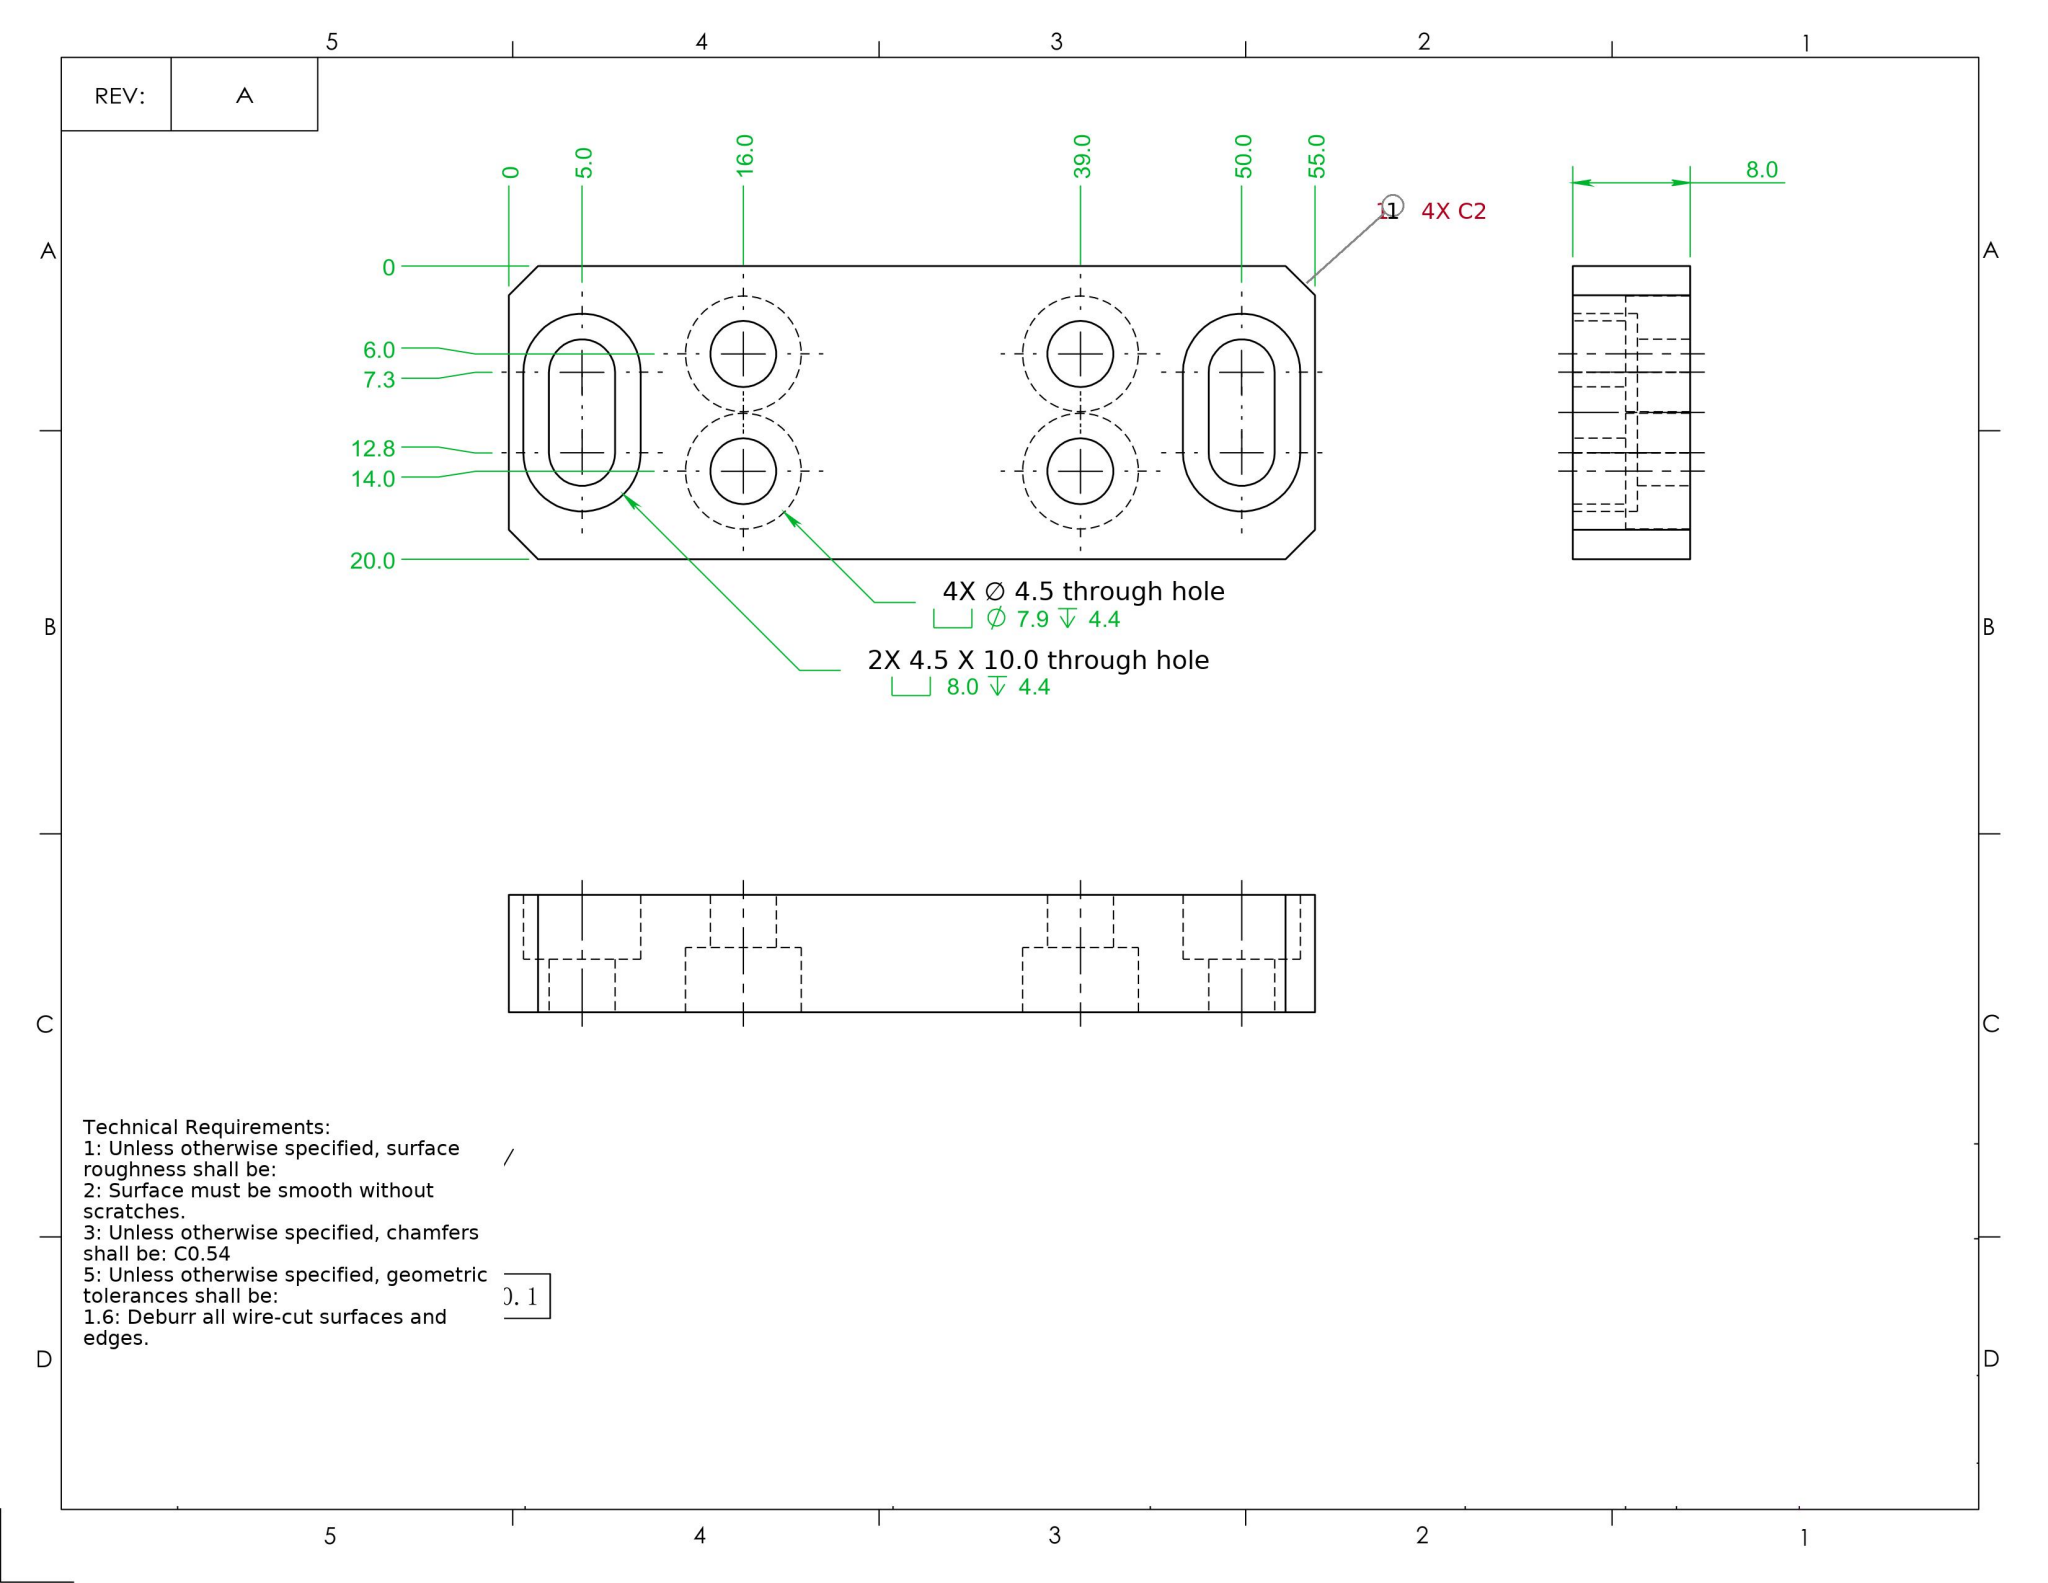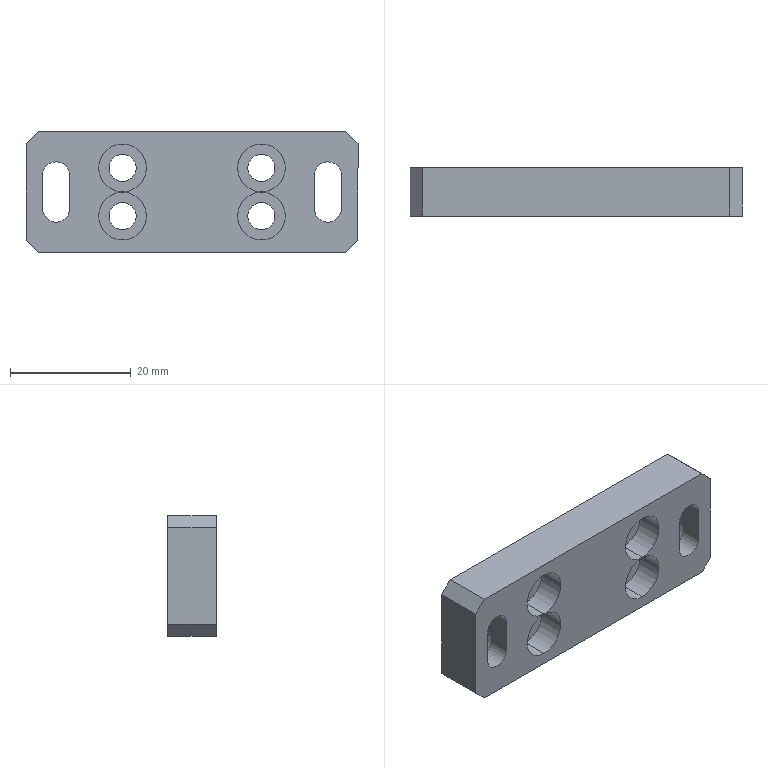Part | SolidWorks | mm | 1 solid | 52 faces | box 55 x 8 x 20 mm | volume 6522 mm3 | cylinder 28 | plane 24 | commonest cylinder face diameters 4.5 x14 7.9 x8 8 x6